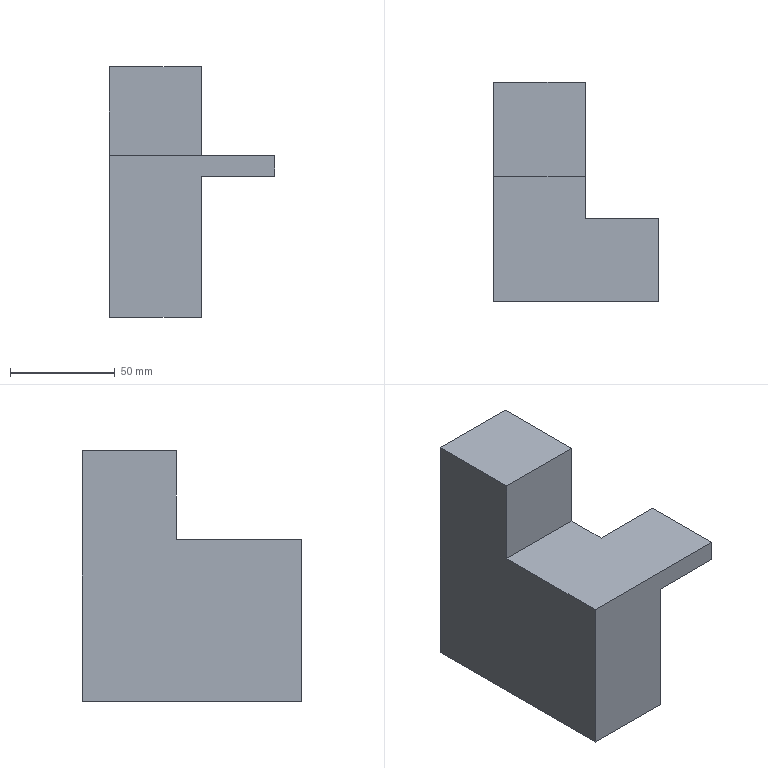Component | SolidWorks | HZ022-A001-E009-1 | 1 solid | 11 faces | box 79 x 105 x 120 mm | volume 456200 mm3 | plane 11 | material AL6061
build123d program:
from build123d import *

# Parameters (mm, degrees)
SKETCH1_W           = 44
SKETCH1_H           = 120
BOSS_EXTRUDE1_DEPTH = 105
SKETCH2_W           = 42.5
SKETCH2_H           = 60
CUT_EXTRUDE1_DEPTH  = 129.69
SKETCH3_W           = 35
SKETCH3_H           = 40
BOSS_EXTRUDE2_DEPTH = 10


with BuildPart() as part:
    # Sketch1 → Boss-Extrude1 (new body)
    with BuildSketch(Plane(origin=(0, 0, 0), x_dir=(1, 0, 0), z_dir=(0, 1, 0))):
        Rectangle(SKETCH1_W, SKETCH1_H)
    extrude(amount=BOSS_EXTRUDE1_DEPTH)

    # Sketch2 → Cut-Extrude1 (cut, through all)
    with BuildSketch(Plane(origin=(22, 0, 0), x_dir=(0, 0, -1), z_dir=(1, 0, 0))):
        with Locations((-38.75, 30)):
            Rectangle(SKETCH2_W, SKETCH2_H)
    extrude(amount=-CUT_EXTRUDE1_DEPTH, mode=Mode.SUBTRACT)

    # Sketch3 → Boss-Extrude2 (add)
    with BuildSketch(Plane.XY.offset(17.5)):
        with Locations((39.5, 20)):
            Rectangle(SKETCH3_W, SKETCH3_H)
    extrude(amount=-BOSS_EXTRUDE2_DEPTH)


solid = part.part

# Placed as in the assembly
solid = solid.moved(Location((153.744, 44.652, 807.5), (0, 0, 0)))
STEP:
#1=COLOUR_RGB('',0.7922,0.8196,0.9333);
#2=FILL_AREA_STYLE_COLOUR('',#1);
#3=FILL_AREA_STYLE('',(#2));
#4=SURFACE_STYLE_FILL_AREA(#3);
#5=SURFACE_SIDE_STYLE('',(#4));
#6=SURFACE_STYLE_USAGE(.BOTH.,#5);
#7=PRESENTATION_STYLE_ASSIGNMENT((#6));
#8=CARTESIAN_POINT('',(6.919,3.333,32.087));
#9=VERTEX_POINT('',#8);
#10=CARTESIAN_POINT('',(6.919,3.333,32.48));
#11=VERTEX_POINT('',#10);
#12=CARTESIAN_POINT('',(6.919,3.333,32.087));
#13=DIRECTION('',(0.,0.,1.));
#14=VECTOR('',#13,39.37);
#15=LINE('',#12,#14);
#16=EDGE_CURVE('',#9,#11,#15,.T.);
#17=ORIENTED_EDGE('',*,*,#16,.F.);
#18=CARTESIAN_POINT('',(6.919,1.758,32.087));
#19=VERTEX_POINT('',#18);
#20=CARTESIAN_POINT('',(6.919,1.758,32.087));
#21=DIRECTION('',(0.,-1.,0.));
#22=VECTOR('',#21,39.37);
#23=LINE('',#20,#22);
#24=EDGE_CURVE('',#9,#19,#23,.T.);
#25=ORIENTED_EDGE('',*,*,#24,.T.);
#26=CARTESIAN_POINT('',(6.919,1.758,29.429));
#27=VERTEX_POINT('',#26);
#28=CARTESIAN_POINT('',(6.919,1.758,29.429));
#29=DIRECTION('',(-0.,0.,-1.));
#30=VECTOR('',#29,39.37);
#31=LINE('',#28,#30);
#32=EDGE_CURVE('',#19,#27,#31,.T.);
#33=ORIENTED_EDGE('',*,*,#32,.T.);
#34=CARTESIAN_POINT('',(6.919,5.892,29.429));
#35=VERTEX_POINT('',#34);
#36=CARTESIAN_POINT('',(6.919,5.892,29.429));
#37=DIRECTION('',(0.,-1.,0.));
#38=VECTOR('',#37,39.37);
#39=LINE('',#36,#38);
#40=EDGE_CURVE('',#35,#27,#39,.T.);
#41=ORIENTED_EDGE('',*,*,#40,.F.);
#42=CARTESIAN_POINT('',(6.919,5.892,34.154));
#43=VERTEX_POINT('',#42);
#44=CARTESIAN_POINT('',(6.919,5.892,29.429));
#45=DIRECTION('',(-0.,0.,-1.));
#46=VECTOR('',#45,39.37);
#47=LINE('',#44,#46);
#48=EDGE_CURVE('',#43,#35,#47,.T.);
#49=ORIENTED_EDGE('',*,*,#48,.F.);
#50=CARTESIAN_POINT('',(6.919,4.12,34.154));
#51=VERTEX_POINT('',#50);
#52=CARTESIAN_POINT('',(6.919,5.892,34.154));
#53=DIRECTION('',(0.,-1.,0.));
#54=VECTOR('',#53,39.37);
#55=LINE('',#52,#54);
#56=EDGE_CURVE('',#43,#51,#55,.T.);
#57=ORIENTED_EDGE('',*,*,#56,.T.);
#58=CARTESIAN_POINT('',(6.919,4.12,32.48));
#59=VERTEX_POINT('',#58);
#60=CARTESIAN_POINT('',(6.919,4.12,34.154));
#61=DIRECTION('',(0.,0.,1.));
#62=VECTOR('',#61,39.37);
#63=LINE('',#60,#62);
#64=EDGE_CURVE('',#59,#51,#63,.T.);
#65=ORIENTED_EDGE('',*,*,#64,.F.);
#66=CARTESIAN_POINT('',(6.919,1.758,32.48));
#67=DIRECTION('',(0.,1.,0.));
#68=VECTOR('',#67,39.37);
#69=LINE('',#66,#68);
#70=EDGE_CURVE('',#11,#59,#69,.T.);
#71=ORIENTED_EDGE('',*,*,#70,.F.);
#72=EDGE_LOOP('',(#17,#25,#33,#41,#49,#57,#65,#71));
#73=FACE_OUTER_BOUND('',#72,.T.);
#74=CARTESIAN_POINT('',(6.919,5.892,29.429));
#75=DIRECTION('',(-1.,0.,0.));
#76=DIRECTION('',(0.,0.,1.));
#77=AXIS2_PLACEMENT_3D('',#74,#75,#76);
#78=PLANE('',#77);
#79=ADVANCED_FACE('',(#73),#78,.F.);
#80=CARTESIAN_POINT('',(5.187,1.758,29.429));
#81=VERTEX_POINT('',#80);
#82=CARTESIAN_POINT('',(5.187,1.758,29.429));
#83=DIRECTION('',(-1.,0.,0.));
#84=VECTOR('',#83,39.37);
#85=LINE('',#82,#84);
#86=EDGE_CURVE('',#27,#81,#85,.T.);
#87=ORIENTED_EDGE('',*,*,#86,.T.);
#88=CARTESIAN_POINT('',(5.187,5.892,29.429));
#89=VERTEX_POINT('',#88);
#90=CARTESIAN_POINT('',(5.187,5.892,29.429));
#91=DIRECTION('',(0.,-1.,0.));
#92=VECTOR('',#91,39.37);
#93=LINE('',#90,#92);
#94=EDGE_CURVE('',#89,#81,#93,.T.);
#95=ORIENTED_EDGE('',*,*,#94,.F.);
#96=CARTESIAN_POINT('',(5.187,5.892,29.429));
#97=DIRECTION('',(-1.,0.,0.));
#98=VECTOR('',#97,39.37);
#99=LINE('',#96,#98);
#100=EDGE_CURVE('',#35,#89,#99,.T.);
#101=ORIENTED_EDGE('',*,*,#100,.F.);
#102=ORIENTED_EDGE('',*,*,#40,.T.);
#103=EDGE_LOOP('',(#87,#95,#101,#102));
#104=FACE_OUTER_BOUND('',#103,.T.);
#105=CARTESIAN_POINT('',(5.187,5.892,29.429));
#106=DIRECTION('',(0.,0.,1.));
#107=DIRECTION('',(1.,0.,0.));
#108=AXIS2_PLACEMENT_3D('',#105,#106,#107);
#109=PLANE('',#108);
#110=ADVANCED_FACE('',(#104),#109,.F.);
#111=CARTESIAN_POINT('',(5.187,1.758,32.48));
#112=VERTEX_POINT('',#111);
#113=CARTESIAN_POINT('',(5.187,4.12,32.48));
#114=VERTEX_POINT('',#113);
#115=CARTESIAN_POINT('',(5.187,1.758,32.48));
#116=DIRECTION('',(0.,1.,0.));
#117=VECTOR('',#116,39.37);
#118=LINE('',#115,#117);
#119=EDGE_CURVE('',#112,#114,#118,.T.);
#120=ORIENTED_EDGE('',*,*,#119,.T.);
#121=CARTESIAN_POINT('',(5.187,4.12,34.154));
#122=VERTEX_POINT('',#121);
#123=CARTESIAN_POINT('',(5.187,4.12,34.154));
#124=DIRECTION('',(0.,0.,1.));
#125=VECTOR('',#124,39.37);
#126=LINE('',#123,#125);
#127=EDGE_CURVE('',#114,#122,#126,.T.);
#128=ORIENTED_EDGE('',*,*,#127,.T.);
#129=CARTESIAN_POINT('',(5.187,5.892,34.154));
#130=VERTEX_POINT('',#129);
#131=CARTESIAN_POINT('',(5.187,5.892,34.154));
#132=DIRECTION('',(0.,-1.,0.));
#133=VECTOR('',#132,39.37);
#134=LINE('',#131,#133);
#135=EDGE_CURVE('',#130,#122,#134,.T.);
#136=ORIENTED_EDGE('',*,*,#135,.F.);
#137=CARTESIAN_POINT('',(5.187,5.892,29.429));
#138=DIRECTION('',(0.,0.,1.));
#139=VECTOR('',#138,39.37);
#140=LINE('',#137,#139);
#141=EDGE_CURVE('',#89,#130,#140,.T.);
#142=ORIENTED_EDGE('',*,*,#141,.F.);
#143=ORIENTED_EDGE('',*,*,#94,.T.);
#144=CARTESIAN_POINT('',(5.187,1.758,29.429));
#145=DIRECTION('',(0.,0.,1.));
#146=VECTOR('',#145,39.37);
#147=LINE('',#144,#146);
#148=EDGE_CURVE('',#81,#112,#147,.T.);
#149=ORIENTED_EDGE('',*,*,#148,.T.);
#150=EDGE_LOOP('',(#120,#128,#136,#142,#143,#149));
#151=FACE_OUTER_BOUND('',#150,.T.);
#152=CARTESIAN_POINT('',(5.187,5.892,29.429));
#153=DIRECTION('',(1.,0.,-0.));
#154=DIRECTION('',(-0.,0.,-1.));
#155=AXIS2_PLACEMENT_3D('',#152,#153,#154);
#156=PLANE('',#155);
#157=ADVANCED_FACE('',(#151),#156,.F.);
#158=ORIENTED_EDGE('',*,*,#135,.T.);
#159=CARTESIAN_POINT('',(5.187,4.12,34.154));
#160=DIRECTION('',(1.,0.,-0.));
#161=VECTOR('',#160,39.37);
#162=LINE('',#159,#161);
#163=EDGE_CURVE('',#122,#51,#162,.T.);
#164=ORIENTED_EDGE('',*,*,#163,.T.);
#165=ORIENTED_EDGE('',*,*,#56,.F.);
#166=CARTESIAN_POINT('',(5.187,5.892,34.154));
#167=DIRECTION('',(1.,0.,0.));
#168=VECTOR('',#167,39.37);
#169=LINE('',#166,#168);
#170=EDGE_CURVE('',#130,#43,#169,.T.);
#171=ORIENTED_EDGE('',*,*,#170,.F.);
#172=EDGE_LOOP('',(#158,#164,#165,#171));
#173=FACE_OUTER_BOUND('',#172,.T.);
#174=CARTESIAN_POINT('',(5.187,5.892,34.154));
#175=DIRECTION('',(0.,0.,-1.));
#176=DIRECTION('',(-1.,0.,0.));
#177=AXIS2_PLACEMENT_3D('',#174,#175,#176);
#178=PLANE('',#177);
#179=ADVANCED_FACE('',(#173),#178,.F.);
#180=ORIENTED_EDGE('',*,*,#48,.T.);
#181=ORIENTED_EDGE('',*,*,#100,.T.);
#182=ORIENTED_EDGE('',*,*,#141,.T.);
#183=ORIENTED_EDGE('',*,*,#170,.T.);
#184=EDGE_LOOP('',(#180,#181,#182,#183));
#185=FACE_OUTER_BOUND('',#184,.T.);
#186=CARTESIAN_POINT('',(6.053,5.892,31.791));
#187=DIRECTION('',(0.,1.,0.));
#188=DIRECTION('',(0.,0.,1.));
#189=AXIS2_PLACEMENT_3D('',#186,#187,#188);
#190=PLANE('',#189);
#191=ADVANCED_FACE('',(#185),#190,.T.);
#192=ORIENTED_EDGE('',*,*,#32,.F.);
#193=CARTESIAN_POINT('',(8.297,1.758,32.087));
#194=VERTEX_POINT('',#193);
#195=CARTESIAN_POINT('',(6.919,1.758,32.087));
#196=DIRECTION('',(1.,0.,0.));
#197=VECTOR('',#196,39.37);
#198=LINE('',#195,#197);
#199=EDGE_CURVE('',#19,#194,#198,.T.);
#200=ORIENTED_EDGE('',*,*,#199,.T.);
#201=CARTESIAN_POINT('',(8.297,1.758,32.48));
#202=VERTEX_POINT('',#201);
#203=CARTESIAN_POINT('',(8.297,1.758,32.087));
#204=DIRECTION('',(0.,0.,1.));
#205=VECTOR('',#204,39.37);
#206=LINE('',#203,#205);
#207=EDGE_CURVE('',#194,#202,#206,.T.);
#208=ORIENTED_EDGE('',*,*,#207,.T.);
#209=CARTESIAN_POINT('',(5.187,1.758,32.48));
#210=DIRECTION('',(1.,0.,-0.));
#211=VECTOR('',#210,39.37);
#212=LINE('',#209,#211);
#213=EDGE_CURVE('',#112,#202,#212,.T.);
#214=ORIENTED_EDGE('',*,*,#213,.F.);
#215=ORIENTED_EDGE('',*,*,#148,.F.);
#216=ORIENTED_EDGE('',*,*,#86,.F.);
#217=EDGE_LOOP('',(#192,#200,#208,#214,#215,#216));
#218=FACE_OUTER_BOUND('',#217,.T.);
#219=CARTESIAN_POINT('',(6.053,1.758,31.791));
#220=DIRECTION('',(0.,1.,0.));
#221=DIRECTION('',(0.,0.,1.));
#222=AXIS2_PLACEMENT_3D('',#219,#220,#221);
#223=PLANE('',#222);
#224=ADVANCED_FACE('',(#218),#223,.F.);
#225=ORIENTED_EDGE('',*,*,#64,.T.);
#226=ORIENTED_EDGE('',*,*,#163,.F.);
#227=ORIENTED_EDGE('',*,*,#127,.F.);
#228=CARTESIAN_POINT('',(5.187,4.12,32.48));
#229=DIRECTION('',(1.,0.,-0.));
#230=VECTOR('',#229,39.37);
#231=LINE('',#228,#230);
#232=EDGE_CURVE('',#114,#59,#231,.T.);
#233=ORIENTED_EDGE('',*,*,#232,.T.);
#234=EDGE_LOOP('',(#225,#226,#227,#233));
#235=FACE_OUTER_BOUND('',#234,.T.);
#236=CARTESIAN_POINT('',(5.187,4.12,34.154));
#237=DIRECTION('',(0.,1.,0.));
#238=DIRECTION('',(0.,0.,1.));
#239=AXIS2_PLACEMENT_3D('',#236,#237,#238);
#240=PLANE('',#239);
#241=ADVANCED_FACE('',(#235),#240,.F.);
#242=ORIENTED_EDGE('',*,*,#213,.T.);
#243=CARTESIAN_POINT('',(8.297,3.333,32.48));
#244=VERTEX_POINT('',#243);
#245=CARTESIAN_POINT('',(8.297,1.758,32.48));
#246=DIRECTION('',(0.,1.,0.));
#247=VECTOR('',#246,39.37);
#248=LINE('',#245,#247);
#249=EDGE_CURVE('',#202,#244,#248,.T.);
#250=ORIENTED_EDGE('',*,*,#249,.T.);
#251=CARTESIAN_POINT('',(6.919,3.333,32.48));
#252=DIRECTION('',(-1.,0.,0.));
#253=VECTOR('',#252,39.37);
#254=LINE('',#251,#253);
#255=EDGE_CURVE('',#244,#11,#254,.T.);
#256=ORIENTED_EDGE('',*,*,#255,.T.);
#257=ORIENTED_EDGE('',*,*,#70,.T.);
#258=ORIENTED_EDGE('',*,*,#232,.F.);
#259=ORIENTED_EDGE('',*,*,#119,.F.);
#260=EDGE_LOOP('',(#242,#250,#256,#257,#258,#259));
#261=FACE_OUTER_BOUND('',#260,.T.);
#262=CARTESIAN_POINT('',(5.187,1.758,32.48));
#263=DIRECTION('',(-0.,0.,-1.));
#264=DIRECTION('',(-1.,0.,0.));
#265=AXIS2_PLACEMENT_3D('',#262,#263,#264);
#266=PLANE('',#265);
#267=ADVANCED_FACE('',(#261),#266,.F.);
#268=ORIENTED_EDGE('',*,*,#255,.F.);
#269=CARTESIAN_POINT('',(8.297,3.333,32.087));
#270=VERTEX_POINT('',#269);
#271=CARTESIAN_POINT('',(8.297,3.333,32.087));
#272=DIRECTION('',(0.,0.,1.));
#273=VECTOR('',#272,39.37);
#274=LINE('',#271,#273);
#275=EDGE_CURVE('',#270,#244,#274,.T.);
#276=ORIENTED_EDGE('',*,*,#275,.F.);
#277=CARTESIAN_POINT('',(6.919,3.333,32.087));
#278=DIRECTION('',(-1.,0.,0.));
#279=VECTOR('',#278,39.37);
#280=LINE('',#277,#279);
#281=EDGE_CURVE('',#270,#9,#280,.T.);
#282=ORIENTED_EDGE('',*,*,#281,.T.);
#283=ORIENTED_EDGE('',*,*,#16,.T.);
#284=EDGE_LOOP('',(#268,#276,#282,#283));
#285=FACE_OUTER_BOUND('',#284,.T.);
#286=CARTESIAN_POINT('',(6.919,3.333,32.087));
#287=DIRECTION('',(0.,1.,0.));
#288=DIRECTION('',(0.,0.,1.));
#289=AXIS2_PLACEMENT_3D('',#286,#287,#288);
#290=PLANE('',#289);
#291=ADVANCED_FACE('',(#285),#290,.T.);
#292=ORIENTED_EDGE('',*,*,#249,.F.);
#293=ORIENTED_EDGE('',*,*,#207,.F.);
#294=CARTESIAN_POINT('',(8.297,1.758,32.087));
#295=DIRECTION('',(0.,1.,0.));
#296=VECTOR('',#295,39.37);
#297=LINE('',#294,#296);
#298=EDGE_CURVE('',#194,#270,#297,.T.);
#299=ORIENTED_EDGE('',*,*,#298,.T.);
#300=ORIENTED_EDGE('',*,*,#275,.T.);
#301=EDGE_LOOP('',(#292,#293,#299,#300));
#302=FACE_OUTER_BOUND('',#301,.T.);
#303=CARTESIAN_POINT('',(8.297,1.758,32.087));
#304=DIRECTION('',(1.,0.,0.));
#305=DIRECTION('',(0.,0.,-1.));
#306=AXIS2_PLACEMENT_3D('',#303,#304,#305);
#307=PLANE('',#306);
#308=ADVANCED_FACE('',(#302),#307,.T.);
#309=ORIENTED_EDGE('',*,*,#24,.F.);
#310=ORIENTED_EDGE('',*,*,#281,.F.);
#311=ORIENTED_EDGE('',*,*,#298,.F.);
#312=ORIENTED_EDGE('',*,*,#199,.F.);
#313=EDGE_LOOP('',(#309,#310,#311,#312));
#314=FACE_OUTER_BOUND('',#313,.T.);
#315=CARTESIAN_POINT('',(6.053,1.758,32.087));
#316=DIRECTION('',(0.,0.,-1.));
#317=DIRECTION('',(-1.,0.,0.));
#318=AXIS2_PLACEMENT_3D('',#315,#316,#317);
#319=PLANE('',#318);
#320=ADVANCED_FACE('',(#314),#319,.T.);
#321=CLOSED_SHELL('',(#79,#110,#157,#179,#191,#224,#241,#267,#291,#308,#320));
#322=MANIFOLD_SOLID_BREP('',#321);
#323=STYLED_ITEM('',(#7),#322);
#324=(LENGTH_UNIT()NAMED_UNIT(*)SI_UNIT($,.METRE.));
#325=LENGTH_MEASURE_WITH_UNIT(LENGTH_MEASURE(0.0254),#324);
#326=DIMENSIONAL_EXPONENTS(1.,0.,0.,0.,0.,0.,0.);
#327=(CONVERSION_BASED_UNIT('',#325)LENGTH_UNIT()NAMED_UNIT(#326));
#328=UNCERTAINTY_MEASURE_WITH_UNIT(LENGTH_MEASURE(0.00001),#327,'','');
#329=(NAMED_UNIT(*)PLANE_ANGLE_UNIT()SI_UNIT($,.RADIAN.));
#330=(NAMED_UNIT(*)SI_UNIT($,.STERADIAN.)SOLID_ANGLE_UNIT());
#331=(GEOMETRIC_REPRESENTATION_CONTEXT(3)GLOBAL_UNCERTAINTY_ASSIGNED_CONTEXT((#328))GLOBAL_UNIT_ASSIGNED_CONTEXT((#327,#329,#330))REPRESENTATION_CONTEXT('',''));
#332=MECHANICAL_DESIGN_GEOMETRIC_PRESENTATION_REPRESENTATION('',(#323),#331);
#333=CARTESIAN_POINT('',(0.,0.,0.));
#334=DIRECTION('',(0.,0.,1.));
#335=DIRECTION('',(1.,0.,0.));
#336=AXIS2_PLACEMENT_3D('',#333,#334,#335);
#337=(LENGTH_UNIT()NAMED_UNIT(*)SI_UNIT($,.METRE.));
#338=LENGTH_MEASURE_WITH_UNIT(LENGTH_MEASURE(0.0254),#337);
#339=DIMENSIONAL_EXPONENTS(1.,0.,0.,0.,0.,0.,0.);
#340=(CONVERSION_BASED_UNIT('',#338)LENGTH_UNIT()NAMED_UNIT(#339));
#341=UNCERTAINTY_MEASURE_WITH_UNIT(LENGTH_MEASURE(0.00001),#340,'','');
#342=(NAMED_UNIT(*)PLANE_ANGLE_UNIT()SI_UNIT($,.RADIAN.));
#343=(NAMED_UNIT(*)SI_UNIT($,.STERADIAN.)SOLID_ANGLE_UNIT());
#344=(GEOMETRIC_REPRESENTATION_CONTEXT(3)GLOBAL_UNCERTAINTY_ASSIGNED_CONTEXT((#341))GLOBAL_UNIT_ASSIGNED_CONTEXT((#340,#342,#343))REPRESENTATION_CONTEXT('',''));
#345=ADVANCED_BREP_SHAPE_REPRESENTATION('',(#322,#336),#344);
#346=PRESENTATION_LAYER_ASSIGNMENT('','',(#323));